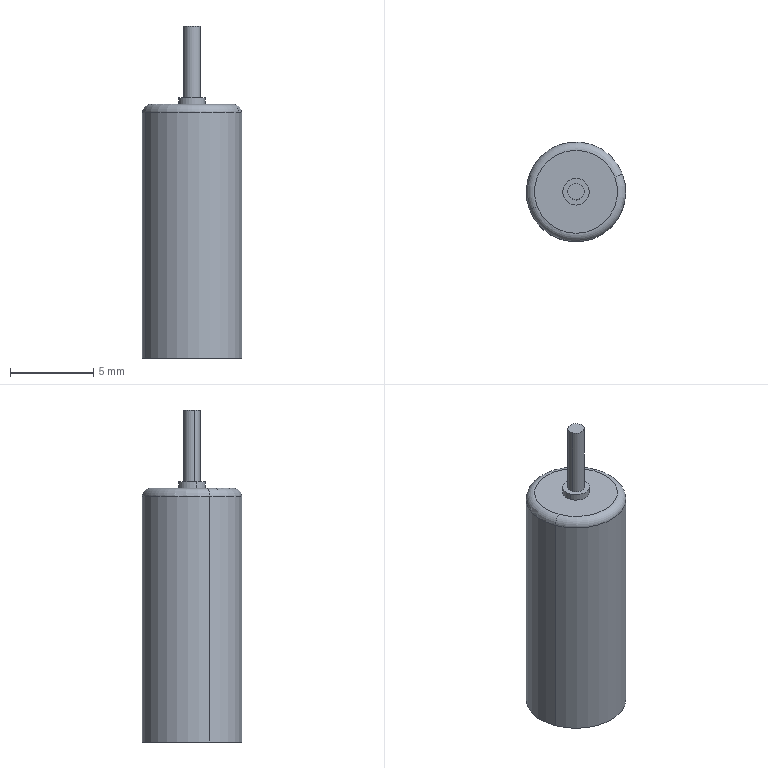Component | SolidWorks | CorelessMotor-1 | 1 solid | 18 faces | box 6 x 6 x 20 mm | volume 434 mm3 | cylinder 10 | plane 6 | torus 2 | commonest cylinder face diameters 1 x6 1.6 x2 6 x2
build123d program:
from build123d import *

# Parameters (mm, degrees)
SKETCH1_R           = 3
BOSS_EXTRUDE1_DEPTH = 15.28
SKETCH3_R           = 0.8
BOSS_EXTRUDE2_DEPTH = 0.4
SKETCH4_R           = 0.5
EXTRUDE_476_DEPTH   = 20
FILLET1_R           = 0.5
SKETCH5_R           = 0.5
CUT_EXTRUDE1_DEPTH  = 0.5


with BuildPart() as part:
    # Sketch1 → Boss-Extrude1 (new body)
    with BuildSketch(Plane.XY):
        with Locations(Location((0, 0, 0), (0, 0, 180))):
            Circle(SKETCH1_R)
    extrude(amount=BOSS_EXTRUDE1_DEPTH)

    # Sketch3 → Boss-Extrude2 (add)
    with BuildSketch(Plane.XY.offset(15.28)):
        Circle(SKETCH3_R)
    extrude(amount=BOSS_EXTRUDE2_DEPTH)

    # Sketch4 → Extrude 476 (add)
    with BuildSketch(Plane(origin=(0, 0, 0), x_dir=(-1, 0, 0), z_dir=(0, 0, -1))):
        Circle(SKETCH4_R)
    extrude(amount=-EXTRUDE_476_DEPTH)

    # Fillet1
    fillet1_edges = [part.edges().sort_by_distance(p)[0] for p in [
        (3, 0, 15.28),
    ]]
    fillet(fillet1_edges, radius=FILLET1_R)

    # Sketch5 → Cut-Extrude1 (cut)
    with BuildSketch(Plane(origin=(0, 0, 0), x_dir=(-1, 0, 0), z_dir=(0, 0, -1))):
        with Locations((-2.4, 0)):
            Circle(SKETCH5_R)
        with Locations((2.4, 0)):
            Circle(SKETCH5_R)
    extrude(amount=-CUT_EXTRUDE1_DEPTH, mode=Mode.SUBTRACT)


solid = part.part

# Placed as in the assembly
solid = solid.moved(Location((0.5486, -2.426, 10.97), (0, 0, 20.828)))
STEP:
#1=COLOUR_RGB('',0.7922,0.8196,0.9333);
#2=FILL_AREA_STYLE_COLOUR('',#1);
#3=FILL_AREA_STYLE('',(#2));
#4=SURFACE_STYLE_FILL_AREA(#3);
#5=SURFACE_SIDE_STYLE('',(#4));
#6=SURFACE_STYLE_USAGE(.BOTH.,#5);
#7=PRESENTATION_STYLE_ASSIGNMENT((#6));
#8=CARTESIAN_POINT('',(-0.08511,-0.1361,0.4516));
#9=VERTEX_POINT('',#8);
#10=CARTESIAN_POINT('',(-0.04832,-0.1221,0.4516));
#11=VERTEX_POINT('',#10);
#12=CARTESIAN_POINT('',(-0.06672,-0.1291,0.4516));
#13=DIRECTION('',(0.,0.,-1.));
#14=DIRECTION('',(0.9347,0.3556,0.));
#15=AXIS2_PLACEMENT_3D('',#12,#13,#14);
#16=CIRCLE('',#15,0.01969);
#17=EDGE_CURVE('',#9,#11,#16,.T.);
#18=ORIENTED_EDGE('',*,*,#17,.F.);
#19=CARTESIAN_POINT('',(-0.08511,-0.1361,0.4319));
#20=VERTEX_POINT('',#19);
#21=CARTESIAN_POINT('',(-0.08511,-0.1361,0.4516));
#22=DIRECTION('',(0.,0.,-1.));
#23=VECTOR('',#22,39.37);
#24=LINE('',#21,#23);
#25=EDGE_CURVE('',#9,#20,#24,.T.);
#26=ORIENTED_EDGE('',*,*,#25,.T.);
#27=CARTESIAN_POINT('',(-0.04832,-0.1221,0.4319));
#28=VERTEX_POINT('',#27);
#29=CARTESIAN_POINT('',(-0.06672,-0.1291,0.4319));
#30=DIRECTION('',(0.,0.,-1.));
#31=DIRECTION('',(0.9347,0.3556,0.));
#32=AXIS2_PLACEMENT_3D('',#29,#30,#31);
#33=CIRCLE('',#32,0.01969);
#34=EDGE_CURVE('',#20,#28,#33,.T.);
#35=ORIENTED_EDGE('',*,*,#34,.T.);
#36=CARTESIAN_POINT('',(-0.04832,-0.1221,0.4516));
#37=DIRECTION('',(0.,0.,-1.));
#38=VECTOR('',#37,39.37);
#39=LINE('',#36,#38);
#40=EDGE_CURVE('',#11,#28,#39,.T.);
#41=ORIENTED_EDGE('',*,*,#40,.F.);
#42=EDGE_LOOP('',(#18,#26,#35,#41));
#43=FACE_OUTER_BOUND('',#42,.T.);
#44=CARTESIAN_POINT('',(-0.06672,-0.1291,0.4516));
#45=DIRECTION('',(0.,0.,-1.));
#46=DIRECTION('',(0.9347,0.3556,0.));
#47=AXIS2_PLACEMENT_3D('',#44,#45,#46);
#48=CYLINDRICAL_SURFACE('',#47,0.01969);
#49=ADVANCED_FACE('',(#43),#48,.F.);
#50=CARTESIAN_POINT('',(0.09151,-0.06891,0.4516));
#51=VERTEX_POINT('',#50);
#52=CARTESIAN_POINT('',(0.1283,-0.05491,0.4516));
#53=VERTEX_POINT('',#52);
#54=CARTESIAN_POINT('',(0.1099,-0.06191,0.4516));
#55=DIRECTION('',(0.,0.,-1.));
#56=DIRECTION('',(0.9347,0.3556,0.));
#57=AXIS2_PLACEMENT_3D('',#54,#55,#56);
#58=CIRCLE('',#57,0.01969);
#59=EDGE_CURVE('',#51,#53,#58,.T.);
#60=ORIENTED_EDGE('',*,*,#59,.F.);
#61=CARTESIAN_POINT('',(0.09151,-0.06891,0.4319));
#62=VERTEX_POINT('',#61);
#63=CARTESIAN_POINT('',(0.09151,-0.06891,0.4516));
#64=DIRECTION('',(0.,0.,-1.));
#65=VECTOR('',#64,39.37);
#66=LINE('',#63,#65);
#67=EDGE_CURVE('',#51,#62,#66,.T.);
#68=ORIENTED_EDGE('',*,*,#67,.T.);
#69=CARTESIAN_POINT('',(0.1283,-0.05491,0.4319));
#70=VERTEX_POINT('',#69);
#71=CARTESIAN_POINT('',(0.1099,-0.06191,0.4319));
#72=DIRECTION('',(0.,0.,-1.));
#73=DIRECTION('',(0.9347,0.3556,0.));
#74=AXIS2_PLACEMENT_3D('',#71,#72,#73);
#75=CIRCLE('',#74,0.01969);
#76=EDGE_CURVE('',#62,#70,#75,.T.);
#77=ORIENTED_EDGE('',*,*,#76,.T.);
#78=CARTESIAN_POINT('',(0.1283,-0.05491,0.4516));
#79=DIRECTION('',(0.,0.,-1.));
#80=VECTOR('',#79,39.37);
#81=LINE('',#78,#80);
#82=EDGE_CURVE('',#53,#70,#81,.T.);
#83=ORIENTED_EDGE('',*,*,#82,.F.);
#84=EDGE_LOOP('',(#60,#68,#77,#83));
#85=FACE_OUTER_BOUND('',#84,.T.);
#86=CARTESIAN_POINT('',(0.1099,-0.06191,0.4516));
#87=DIRECTION('',(0.,0.,-1.));
#88=DIRECTION('',(0.9347,0.3556,0.));
#89=AXIS2_PLACEMENT_3D('',#86,#87,#88);
#90=CYLINDRICAL_SURFACE('',#89,0.01969);
#91=ADVANCED_FACE('',(#85),#90,.F.);
#92=CARTESIAN_POINT('',(0.132,-0.05351,1.014));
#93=VERTEX_POINT('',#92);
#94=CARTESIAN_POINT('',(-0.08879,-0.1375,1.014));
#95=VERTEX_POINT('',#94);
#96=CARTESIAN_POINT('',(0.0216,-0.0955,1.014));
#97=DIRECTION('',(0.,0.,-1.));
#98=DIRECTION('',(-0.9347,-0.3556,0.));
#99=AXIS2_PLACEMENT_3D('',#96,#97,#98);
#100=CIRCLE('',#99,0.1181);
#101=EDGE_CURVE('',#93,#95,#100,.T.);
#102=ORIENTED_EDGE('',*,*,#101,.F.);
#103=CARTESIAN_POINT('',(0.1136,-0.06051,1.033));
#104=VERTEX_POINT('',#103);
#105=CARTESIAN_POINT('',(0.1136,-0.06051,1.014));
#106=DIRECTION('',(0.3556,-0.9347,0.));
#107=DIRECTION('',(0.9347,0.3556,0.));
#108=AXIS2_PLACEMENT_3D('',#105,#106,#107);
#109=CIRCLE('',#108,0.01969);
#110=EDGE_CURVE('',#93,#104,#109,.T.);
#111=ORIENTED_EDGE('',*,*,#110,.T.);
#112=CARTESIAN_POINT('',(-0.07039,-0.1305,1.033));
#113=VERTEX_POINT('',#112);
#114=CARTESIAN_POINT('',(0.0216,-0.0955,1.033));
#115=DIRECTION('',(0.,0.,1.));
#116=DIRECTION('',(-0.9347,-0.3556,0.));
#117=AXIS2_PLACEMENT_3D('',#114,#115,#116);
#118=CIRCLE('',#117,0.09843);
#119=EDGE_CURVE('',#113,#104,#118,.T.);
#120=ORIENTED_EDGE('',*,*,#119,.F.);
#121=CARTESIAN_POINT('',(-0.07039,-0.1305,1.014));
#122=DIRECTION('',(-0.3556,0.9347,0.));
#123=DIRECTION('',(-0.9347,-0.3556,0.));
#124=AXIS2_PLACEMENT_3D('',#121,#122,#123);
#125=CIRCLE('',#124,0.01969);
#126=EDGE_CURVE('',#95,#113,#125,.T.);
#127=ORIENTED_EDGE('',*,*,#126,.F.);
#128=EDGE_LOOP('',(#102,#111,#120,#127));
#129=FACE_OUTER_BOUND('',#128,.T.);
#130=CARTESIAN_POINT('',(0.0216,-0.0955,1.014));
#131=DIRECTION('',(0.,0.,1.));
#132=DIRECTION('',(-0.9347,-0.3556,0.));
#133=AXIS2_PLACEMENT_3D('',#130,#131,#132);
#134=TOROIDAL_SURFACE('',#133,0.09843,0.01969);
#135=ADVANCED_FACE('',(#129),#134,.T.);
#136=CARTESIAN_POINT('',(0.04,-0.0885,1.219));
#137=VERTEX_POINT('',#136);
#138=CARTESIAN_POINT('',(0.0032,-0.1025,1.219));
#139=VERTEX_POINT('',#138);
#140=CARTESIAN_POINT('',(0.0216,-0.0955,1.219));
#141=DIRECTION('',(0.,0.,-1.));
#142=DIRECTION('',(0.9347,0.3556,0.));
#143=AXIS2_PLACEMENT_3D('',#140,#141,#142);
#144=CIRCLE('',#143,0.01969);
#145=EDGE_CURVE('',#137,#139,#144,.T.);
#146=ORIENTED_EDGE('',*,*,#145,.T.);
#147=CARTESIAN_POINT('',(0.0032,-0.1025,1.049));
#148=VERTEX_POINT('',#147);
#149=CARTESIAN_POINT('',(0.0032,-0.1025,1.219));
#150=DIRECTION('',(0.,0.,-1.));
#151=VECTOR('',#150,39.37);
#152=LINE('',#149,#151);
#153=EDGE_CURVE('',#139,#148,#152,.T.);
#154=ORIENTED_EDGE('',*,*,#153,.T.);
#155=CARTESIAN_POINT('',(0.04,-0.0885,1.049));
#156=VERTEX_POINT('',#155);
#157=CARTESIAN_POINT('',(0.0216,-0.0955,1.049));
#158=DIRECTION('',(0.,0.,1.));
#159=DIRECTION('',(-0.9347,-0.3556,0.));
#160=AXIS2_PLACEMENT_3D('',#157,#158,#159);
#161=CIRCLE('',#160,0.01969);
#162=EDGE_CURVE('',#148,#156,#161,.T.);
#163=ORIENTED_EDGE('',*,*,#162,.T.);
#164=CARTESIAN_POINT('',(0.04,-0.0885,1.219));
#165=DIRECTION('',(0.,0.,-1.));
#166=VECTOR('',#165,39.37);
#167=LINE('',#164,#166);
#168=EDGE_CURVE('',#137,#156,#167,.T.);
#169=ORIENTED_EDGE('',*,*,#168,.F.);
#170=EDGE_LOOP('',(#146,#154,#163,#169));
#171=FACE_OUTER_BOUND('',#170,.T.);
#172=CARTESIAN_POINT('',(0.0216,-0.0955,1.219));
#173=DIRECTION('',(0.,0.,-1.));
#174=DIRECTION('',(0.9347,0.3556,0.));
#175=AXIS2_PLACEMENT_3D('',#172,#173,#174);
#176=CYLINDRICAL_SURFACE('',#175,0.01969);
#177=ADVANCED_FACE('',(#171),#176,.T.);
#178=CARTESIAN_POINT('',(-0.007839,-0.1067,1.049));
#179=VERTEX_POINT('',#178);
#180=CARTESIAN_POINT('',(0.05104,-0.08431,1.049));
#181=VERTEX_POINT('',#180);
#182=CARTESIAN_POINT('',(0.0216,-0.0955,1.049));
#183=DIRECTION('',(0.,0.,1.));
#184=DIRECTION('',(-0.9347,-0.3556,0.));
#185=AXIS2_PLACEMENT_3D('',#182,#183,#184);
#186=CIRCLE('',#185,0.0315);
#187=EDGE_CURVE('',#179,#181,#186,.T.);
#188=ORIENTED_EDGE('',*,*,#187,.F.);
#189=CARTESIAN_POINT('',(-0.007839,-0.1067,1.033));
#190=VERTEX_POINT('',#189);
#191=CARTESIAN_POINT('',(-0.007839,-0.1067,1.049));
#192=DIRECTION('',(0.,0.,-1.));
#193=VECTOR('',#192,39.37);
#194=LINE('',#191,#193);
#195=EDGE_CURVE('',#179,#190,#194,.T.);
#196=ORIENTED_EDGE('',*,*,#195,.T.);
#197=CARTESIAN_POINT('',(0.05104,-0.08431,1.033));
#198=VERTEX_POINT('',#197);
#199=CARTESIAN_POINT('',(0.0216,-0.0955,1.033));
#200=DIRECTION('',(0.,0.,1.));
#201=DIRECTION('',(-0.9347,-0.3556,0.));
#202=AXIS2_PLACEMENT_3D('',#199,#200,#201);
#203=CIRCLE('',#202,0.0315);
#204=EDGE_CURVE('',#190,#198,#203,.T.);
#205=ORIENTED_EDGE('',*,*,#204,.T.);
#206=CARTESIAN_POINT('',(0.05104,-0.08431,1.049));
#207=DIRECTION('',(0.,0.,-1.));
#208=VECTOR('',#207,39.37);
#209=LINE('',#206,#208);
#210=EDGE_CURVE('',#181,#198,#209,.T.);
#211=ORIENTED_EDGE('',*,*,#210,.F.);
#212=EDGE_LOOP('',(#188,#196,#205,#211));
#213=FACE_OUTER_BOUND('',#212,.T.);
#214=CARTESIAN_POINT('',(0.0216,-0.0955,1.049));
#215=DIRECTION('',(0.,0.,-1.));
#216=DIRECTION('',(0.9347,0.3556,0.));
#217=AXIS2_PLACEMENT_3D('',#214,#215,#216);
#218=CYLINDRICAL_SURFACE('',#217,0.0315);
#219=ADVANCED_FACE('',(#213),#218,.T.);
#220=ORIENTED_EDGE('',*,*,#101,.T.);
#221=CARTESIAN_POINT('',(-0.08879,-0.1375,0.4319));
#222=VERTEX_POINT('',#221);
#223=CARTESIAN_POINT('',(-0.08879,-0.1375,1.033));
#224=DIRECTION('',(0.,0.,-1.));
#225=VECTOR('',#224,39.37);
#226=LINE('',#223,#225);
#227=EDGE_CURVE('',#95,#222,#226,.T.);
#228=ORIENTED_EDGE('',*,*,#227,.T.);
#229=CARTESIAN_POINT('',(0.132,-0.05351,0.4319));
#230=VERTEX_POINT('',#229);
#231=CARTESIAN_POINT('',(0.0216,-0.0955,0.4319));
#232=DIRECTION('',(0.,0.,1.));
#233=DIRECTION('',(-0.9347,-0.3556,0.));
#234=AXIS2_PLACEMENT_3D('',#231,#232,#233);
#235=CIRCLE('',#234,0.1181);
#236=EDGE_CURVE('',#222,#230,#235,.T.);
#237=ORIENTED_EDGE('',*,*,#236,.T.);
#238=CARTESIAN_POINT('',(0.132,-0.05351,1.033));
#239=DIRECTION('',(0.,0.,-1.));
#240=VECTOR('',#239,39.37);
#241=LINE('',#238,#240);
#242=EDGE_CURVE('',#93,#230,#241,.T.);
#243=ORIENTED_EDGE('',*,*,#242,.F.);
#244=EDGE_LOOP('',(#220,#228,#237,#243));
#245=FACE_OUTER_BOUND('',#244,.T.);
#246=CARTESIAN_POINT('',(0.0216,-0.0955,1.033));
#247=DIRECTION('',(0.,0.,-1.));
#248=DIRECTION('',(0.9347,0.3556,0.));
#249=AXIS2_PLACEMENT_3D('',#246,#247,#248);
#250=CYLINDRICAL_SURFACE('',#249,0.1181);
#251=ADVANCED_FACE('',(#245),#250,.T.);
#252=ORIENTED_EDGE('',*,*,#227,.F.);
#253=CARTESIAN_POINT('',(0.0216,-0.0955,1.014));
#254=DIRECTION('',(0.,0.,-1.));
#255=DIRECTION('',(-0.9347,-0.3556,0.));
#256=AXIS2_PLACEMENT_3D('',#253,#254,#255);
#257=CIRCLE('',#256,0.1181);
#258=EDGE_CURVE('',#95,#93,#257,.T.);
#259=ORIENTED_EDGE('',*,*,#258,.T.);
#260=ORIENTED_EDGE('',*,*,#242,.T.);
#261=CARTESIAN_POINT('',(0.0216,-0.0955,0.4319));
#262=DIRECTION('',(0.,0.,1.));
#263=DIRECTION('',(-0.9347,-0.3556,0.));
#264=AXIS2_PLACEMENT_3D('',#261,#262,#263);
#265=CIRCLE('',#264,0.1181);
#266=EDGE_CURVE('',#230,#222,#265,.T.);
#267=ORIENTED_EDGE('',*,*,#266,.T.);
#268=EDGE_LOOP('',(#252,#259,#260,#267));
#269=FACE_OUTER_BOUND('',#268,.T.);
#270=CARTESIAN_POINT('',(0.0216,-0.0955,1.033));
#271=DIRECTION('',(0.,0.,-1.));
#272=DIRECTION('',(0.9347,0.3556,0.));
#273=AXIS2_PLACEMENT_3D('',#270,#271,#272);
#274=CYLINDRICAL_SURFACE('',#273,0.1181);
#275=ADVANCED_FACE('',(#269),#274,.T.);
#276=ORIENTED_EDGE('',*,*,#119,.T.);
#277=CARTESIAN_POINT('',(0.0216,-0.0955,1.033));
#278=DIRECTION('',(0.,0.,1.));
#279=DIRECTION('',(-0.9347,-0.3556,0.));
#280=AXIS2_PLACEMENT_3D('',#277,#278,#279);
#281=CIRCLE('',#280,0.09843);
#282=EDGE_CURVE('',#104,#113,#281,.T.);
#283=ORIENTED_EDGE('',*,*,#282,.T.);
#284=EDGE_LOOP('',(#276,#283));
#285=FACE_OUTER_BOUND('',#284,.T.);
#286=CARTESIAN_POINT('',(0.0216,-0.0955,1.033));
#287=DIRECTION('',(0.,0.,1.));
#288=DIRECTION('',(-0.9347,-0.3556,0.));
#289=AXIS2_PLACEMENT_3D('',#286,#287,#288);
#290=CIRCLE('',#289,0.0315);
#291=EDGE_CURVE('',#198,#190,#290,.T.);
#292=ORIENTED_EDGE('',*,*,#291,.F.);
#293=ORIENTED_EDGE('',*,*,#204,.F.);
#294=EDGE_LOOP('',(#292,#293));
#295=FACE_BOUND('',#294,.T.);
#296=CARTESIAN_POINT('',(0.0216,-0.0955,1.033));
#297=DIRECTION('',(0.,0.,1.));
#298=DIRECTION('',(-0.9347,-0.3556,0.));
#299=AXIS2_PLACEMENT_3D('',#296,#297,#298);
#300=PLANE('',#299);
#301=ADVANCED_FACE('',(#285,#295),#300,.T.);
#302=CARTESIAN_POINT('',(-0.06672,-0.1291,0.4319));
#303=DIRECTION('',(0.,0.,-1.));
#304=DIRECTION('',(0.9347,0.3556,0.));
#305=AXIS2_PLACEMENT_3D('',#302,#303,#304);
#306=CIRCLE('',#305,0.01969);
#307=EDGE_CURVE('',#28,#20,#306,.T.);
#308=ORIENTED_EDGE('',*,*,#307,.F.);
#309=ORIENTED_EDGE('',*,*,#34,.F.);
#310=EDGE_LOOP('',(#308,#309));
#311=FACE_BOUND('',#310,.T.);
#312=CARTESIAN_POINT('',(0.1099,-0.06191,0.4319));
#313=DIRECTION('',(0.,0.,-1.));
#314=DIRECTION('',(0.9347,0.3556,0.));
#315=AXIS2_PLACEMENT_3D('',#312,#313,#314);
#316=CIRCLE('',#315,0.01969);
#317=EDGE_CURVE('',#70,#62,#316,.T.);
#318=ORIENTED_EDGE('',*,*,#317,.F.);
#319=ORIENTED_EDGE('',*,*,#76,.F.);
#320=EDGE_LOOP('',(#318,#319));
#321=FACE_BOUND('',#320,.T.);
#322=ORIENTED_EDGE('',*,*,#266,.F.);
#323=ORIENTED_EDGE('',*,*,#236,.F.);
#324=EDGE_LOOP('',(#322,#323));
#325=FACE_OUTER_BOUND('',#324,.T.);
#326=CARTESIAN_POINT('',(0.0216,-0.0955,0.4319));
#327=DIRECTION('',(0.,0.,1.));
#328=DIRECTION('',(-0.9347,-0.3556,0.));
#329=AXIS2_PLACEMENT_3D('',#326,#327,#328);
#330=PLANE('',#329);
#331=ADVANCED_FACE('',(#311,#321,#325),#330,.F.);
#332=ORIENTED_EDGE('',*,*,#195,.F.);
#333=CARTESIAN_POINT('',(0.0216,-0.0955,1.049));
#334=DIRECTION('',(0.,0.,1.));
#335=DIRECTION('',(-0.9347,-0.3556,0.));
#336=AXIS2_PLACEMENT_3D('',#333,#334,#335);
#337=CIRCLE('',#336,0.0315);
#338=EDGE_CURVE('',#181,#179,#337,.T.);
#339=ORIENTED_EDGE('',*,*,#338,.F.);
#340=ORIENTED_EDGE('',*,*,#210,.T.);
#341=ORIENTED_EDGE('',*,*,#291,.T.);
#342=EDGE_LOOP('',(#332,#339,#340,#341));
#343=FACE_OUTER_BOUND('',#342,.T.);
#344=CARTESIAN_POINT('',(0.0216,-0.0955,1.049));
#345=DIRECTION('',(0.,0.,-1.));
#346=DIRECTION('',(0.9347,0.3556,0.));
#347=AXIS2_PLACEMENT_3D('',#344,#345,#346);
#348=CYLINDRICAL_SURFACE('',#347,0.0315);
#349=ADVANCED_FACE('',(#343),#348,.T.);
#350=CARTESIAN_POINT('',(0.0216,-0.0955,1.049));
#351=DIRECTION('',(0.,0.,1.));
#352=DIRECTION('',(-0.9347,-0.3556,0.));
#353=AXIS2_PLACEMENT_3D('',#350,#351,#352);
#354=CIRCLE('',#353,0.01969);
#355=EDGE_CURVE('',#156,#148,#354,.T.);
#356=ORIENTED_EDGE('',*,*,#355,.F.);
#357=ORIENTED_EDGE('',*,*,#162,.F.);
#358=EDGE_LOOP('',(#356,#357));
#359=FACE_BOUND('',#358,.T.);
#360=ORIENTED_EDGE('',*,*,#338,.T.);
#361=ORIENTED_EDGE('',*,*,#187,.T.);
#362=EDGE_LOOP('',(#360,#361));
#363=FACE_OUTER_BOUND('',#362,.T.);
#364=CARTESIAN_POINT('',(0.0216,-0.0955,1.049));
#365=DIRECTION('',(0.,0.,1.));
#366=DIRECTION('',(-0.9347,-0.3556,0.));
#367=AXIS2_PLACEMENT_3D('',#364,#365,#366);
#368=PLANE('',#367);
#369=ADVANCED_FACE('',(#359,#363),#368,.T.);
#370=ORIENTED_EDGE('',*,*,#153,.F.);
#371=CARTESIAN_POINT('',(0.0216,-0.0955,1.219));
#372=DIRECTION('',(0.,0.,-1.));
#373=DIRECTION('',(0.9347,0.3556,0.));
#374=AXIS2_PLACEMENT_3D('',#371,#372,#373);
#375=CIRCLE('',#374,0.01969);
#376=EDGE_CURVE('',#139,#137,#375,.T.);
#377=ORIENTED_EDGE('',*,*,#376,.T.);
#378=ORIENTED_EDGE('',*,*,#168,.T.);
#379=ORIENTED_EDGE('',*,*,#355,.T.);
#380=EDGE_LOOP('',(#370,#377,#378,#379));
#381=FACE_OUTER_BOUND('',#380,.T.);
#382=CARTESIAN_POINT('',(0.0216,-0.0955,1.219));
#383=DIRECTION('',(0.,0.,-1.));
#384=DIRECTION('',(0.9347,0.3556,0.));
#385=AXIS2_PLACEMENT_3D('',#382,#383,#384);
#386=CYLINDRICAL_SURFACE('',#385,0.01969);
#387=ADVANCED_FACE('',(#381),#386,.T.);
#388=ORIENTED_EDGE('',*,*,#145,.F.);
#389=ORIENTED_EDGE('',*,*,#376,.F.);
#390=EDGE_LOOP('',(#388,#389));
#391=FACE_OUTER_BOUND('',#390,.T.);
#392=CARTESIAN_POINT('',(0.0216,-0.0955,1.219));
#393=DIRECTION('',(0.,0.,-1.));
#394=DIRECTION('',(0.9347,0.3556,0.));
#395=AXIS2_PLACEMENT_3D('',#392,#393,#394);
#396=PLANE('',#395);
#397=ADVANCED_FACE('',(#391),#396,.F.);
#398=ORIENTED_EDGE('',*,*,#110,.F.);
#399=ORIENTED_EDGE('',*,*,#258,.F.);
#400=ORIENTED_EDGE('',*,*,#126,.T.);
#401=ORIENTED_EDGE('',*,*,#282,.F.);
#402=EDGE_LOOP('',(#398,#399,#400,#401));
#403=FACE_OUTER_BOUND('',#402,.T.);
#404=CARTESIAN_POINT('',(0.0216,-0.0955,1.014));
#405=DIRECTION('',(0.,0.,1.));
#406=DIRECTION('',(-0.9347,-0.3556,0.));
#407=AXIS2_PLACEMENT_3D('',#404,#405,#406);
#408=TOROIDAL_SURFACE('',#407,0.09843,0.01969);
#409=ADVANCED_FACE('',(#403),#408,.T.);
#410=ORIENTED_EDGE('',*,*,#67,.F.);
#411=CARTESIAN_POINT('',(0.1099,-0.06191,0.4516));
#412=DIRECTION('',(0.,0.,-1.));
#413=DIRECTION('',(0.9347,0.3556,0.));
#414=AXIS2_PLACEMENT_3D('',#411,#412,#413);
#415=CIRCLE('',#414,0.01969);
#416=EDGE_CURVE('',#53,#51,#415,.T.);
#417=ORIENTED_EDGE('',*,*,#416,.F.);
#418=ORIENTED_EDGE('',*,*,#82,.T.);
#419=ORIENTED_EDGE('',*,*,#317,.T.);
#420=EDGE_LOOP('',(#410,#417,#418,#419));
#421=FACE_OUTER_BOUND('',#420,.T.);
#422=CARTESIAN_POINT('',(0.1099,-0.06191,0.4516));
#423=DIRECTION('',(0.,0.,-1.));
#424=DIRECTION('',(0.9347,0.3556,0.));
#425=AXIS2_PLACEMENT_3D('',#422,#423,#424);
#426=CYLINDRICAL_SURFACE('',#425,0.01969);
#427=ADVANCED_FACE('',(#421),#426,.F.);
#428=ORIENTED_EDGE('',*,*,#416,.T.);
#429=ORIENTED_EDGE('',*,*,#59,.T.);
#430=EDGE_LOOP('',(#428,#429));
#431=FACE_OUTER_BOUND('',#430,.T.);
#432=CARTESIAN_POINT('',(0.1099,-0.06191,0.4516));
#433=DIRECTION('',(0.,0.,-1.));
#434=DIRECTION('',(0.9347,0.3556,0.));
#435=AXIS2_PLACEMENT_3D('',#432,#433,#434);
#436=PLANE('',#435);
#437=ADVANCED_FACE('',(#431),#436,.T.);
#438=ORIENTED_EDGE('',*,*,#25,.F.);
#439=CARTESIAN_POINT('',(-0.06672,-0.1291,0.4516));
#440=DIRECTION('',(0.,0.,-1.));
#441=DIRECTION('',(0.9347,0.3556,0.));
#442=AXIS2_PLACEMENT_3D('',#439,#440,#441);
#443=CIRCLE('',#442,0.01969);
#444=EDGE_CURVE('',#11,#9,#443,.T.);
#445=ORIENTED_EDGE('',*,*,#444,.F.);
#446=ORIENTED_EDGE('',*,*,#40,.T.);
#447=ORIENTED_EDGE('',*,*,#307,.T.);
#448=EDGE_LOOP('',(#438,#445,#446,#447));
#449=FACE_OUTER_BOUND('',#448,.T.);
#450=CARTESIAN_POINT('',(-0.06672,-0.1291,0.4516));
#451=DIRECTION('',(0.,0.,-1.));
#452=DIRECTION('',(0.9347,0.3556,0.));
#453=AXIS2_PLACEMENT_3D('',#450,#451,#452);
#454=CYLINDRICAL_SURFACE('',#453,0.01969);
#455=ADVANCED_FACE('',(#449),#454,.F.);
#456=ORIENTED_EDGE('',*,*,#444,.T.);
#457=ORIENTED_EDGE('',*,*,#17,.T.);
#458=EDGE_LOOP('',(#456,#457));
#459=FACE_OUTER_BOUND('',#458,.T.);
#460=CARTESIAN_POINT('',(-0.06672,-0.1291,0.4516));
#461=DIRECTION('',(0.,0.,-1.));
#462=DIRECTION('',(0.9347,0.3556,0.));
#463=AXIS2_PLACEMENT_3D('',#460,#461,#462);
#464=PLANE('',#463);
#465=ADVANCED_FACE('',(#459),#464,.T.);
#466=CLOSED_SHELL('',(#49,#91,#135,#177,#219,#251,#275,#301,#331,#349,#369,#387,#397,#409,#427,#437,#455,#465));
#467=MANIFOLD_SOLID_BREP('',#466);
#468=STYLED_ITEM('',(#7),#467);
#469=(LENGTH_UNIT()NAMED_UNIT(*)SI_UNIT($,.METRE.));
#470=LENGTH_MEASURE_WITH_UNIT(LENGTH_MEASURE(0.0254),#469);
#471=DIMENSIONAL_EXPONENTS(1.,0.,0.,0.,0.,0.,0.);
#472=(CONVERSION_BASED_UNIT('',#470)LENGTH_UNIT()NAMED_UNIT(#471));
#473=UNCERTAINTY_MEASURE_WITH_UNIT(LENGTH_MEASURE(0.00001),#472,'','');
#474=(NAMED_UNIT(*)PLANE_ANGLE_UNIT()SI_UNIT($,.RADIAN.));
#475=(NAMED_UNIT(*)SI_UNIT($,.STERADIAN.)SOLID_ANGLE_UNIT());
#476=(GEOMETRIC_REPRESENTATION_CONTEXT(3)GLOBAL_UNCERTAINTY_ASSIGNED_CONTEXT((#473))GLOBAL_UNIT_ASSIGNED_CONTEXT((#472,#474,#475))REPRESENTATION_CONTEXT('',''));
#477=MECHANICAL_DESIGN_GEOMETRIC_PRESENTATION_REPRESENTATION('',(#468),#476);
#478=PRESENTATION_LAYER_ASSIGNMENT('','',(#468));
#479=CARTESIAN_POINT('',(0.,0.,0.));
#480=DIRECTION('',(0.,0.,1.));
#481=DIRECTION('',(1.,0.,0.));
#482=AXIS2_PLACEMENT_3D('',#479,#480,#481);
#483=(LENGTH_UNIT()NAMED_UNIT(*)SI_UNIT($,.METRE.));
#484=LENGTH_MEASURE_WITH_UNIT(LENGTH_MEASURE(0.0254),#483);
#485=DIMENSIONAL_EXPONENTS(1.,0.,0.,0.,0.,0.,0.);
#486=(CONVERSION_BASED_UNIT('',#484)LENGTH_UNIT()NAMED_UNIT(#485));
#487=UNCERTAINTY_MEASURE_WITH_UNIT(LENGTH_MEASURE(0.00001),#486,'','');
#488=(NAMED_UNIT(*)PLANE_ANGLE_UNIT()SI_UNIT($,.RADIAN.));
#489=(NAMED_UNIT(*)SI_UNIT($,.STERADIAN.)SOLID_ANGLE_UNIT());
#490=(GEOMETRIC_REPRESENTATION_CONTEXT(3)GLOBAL_UNCERTAINTY_ASSIGNED_CONTEXT((#487))GLOBAL_UNIT_ASSIGNED_CONTEXT((#486,#488,#489))REPRESENTATION_CONTEXT('',''));
#491=ADVANCED_BREP_SHAPE_REPRESENTATION('',(#467,#482),#490);